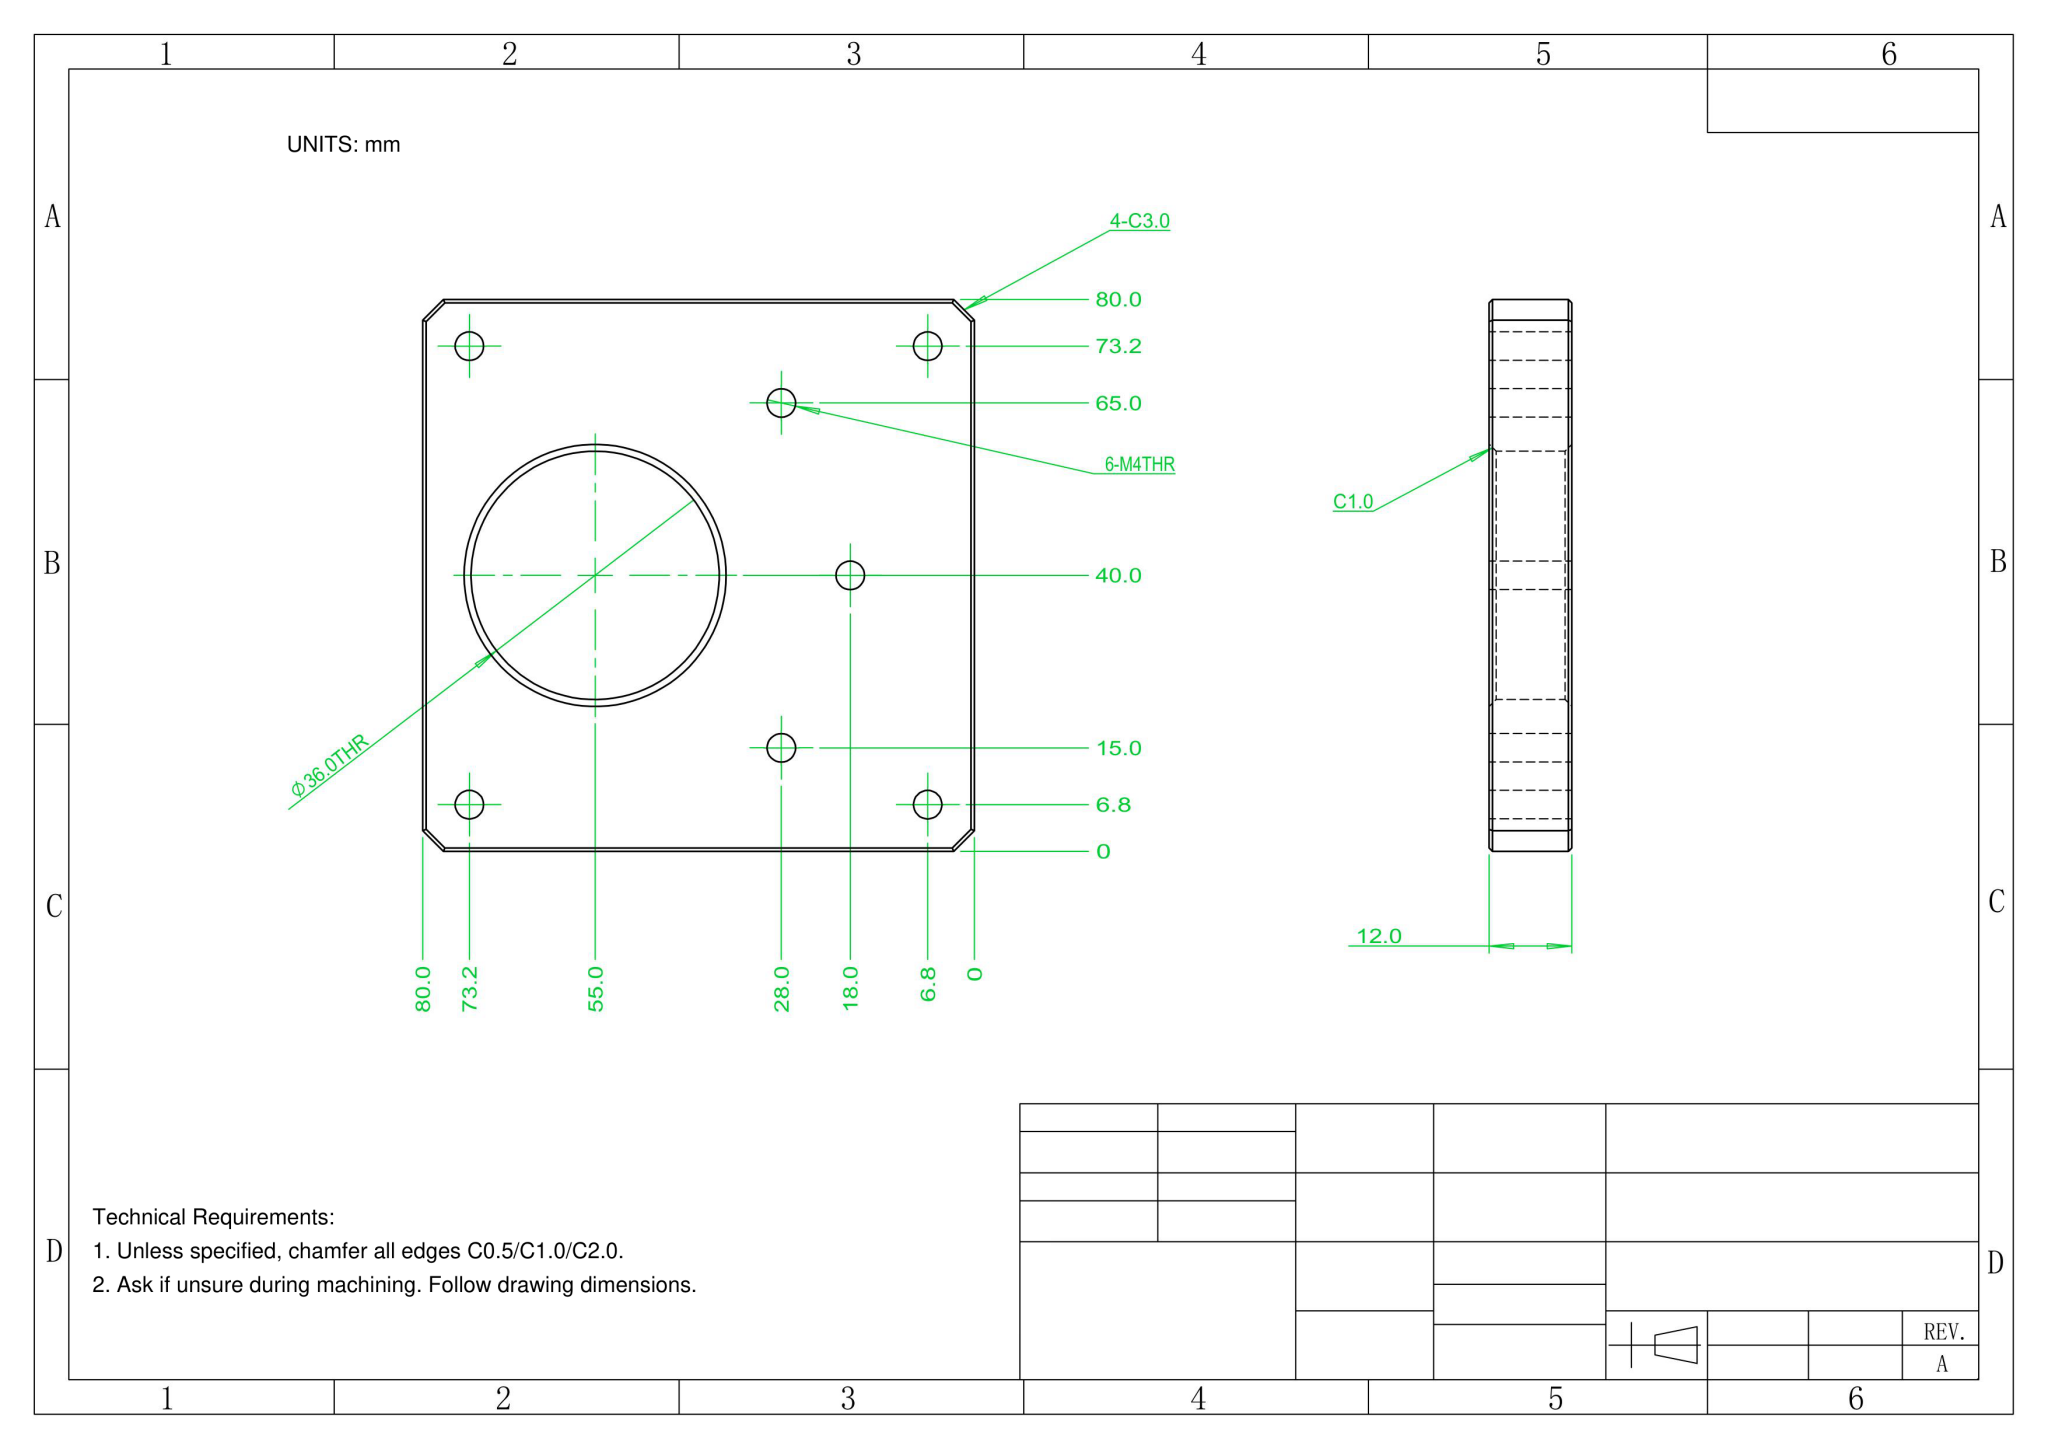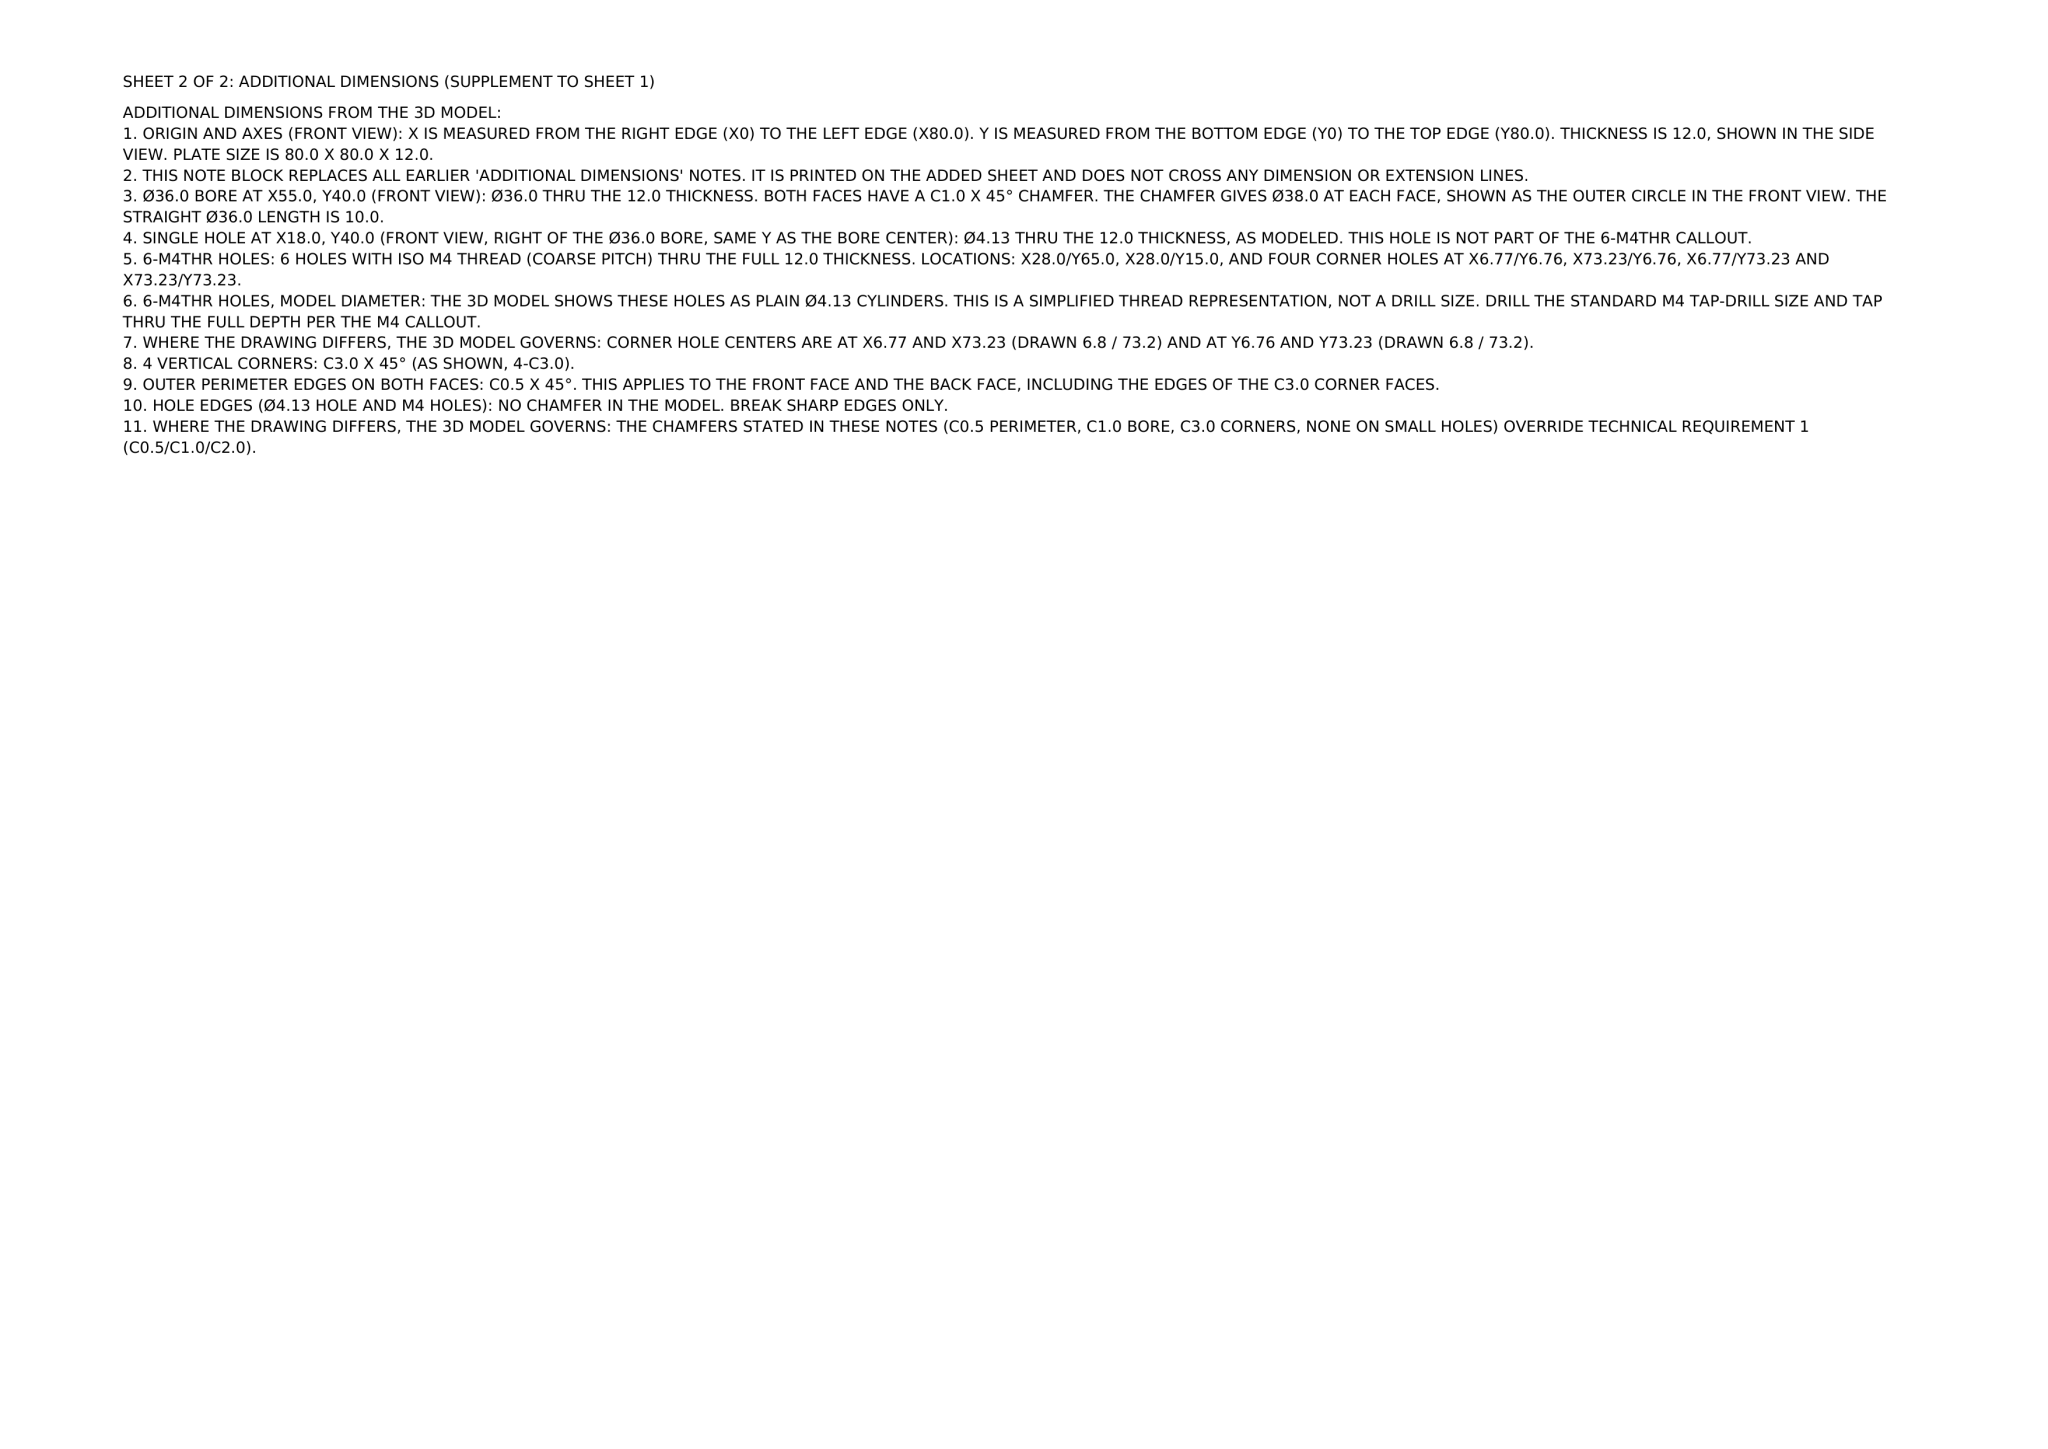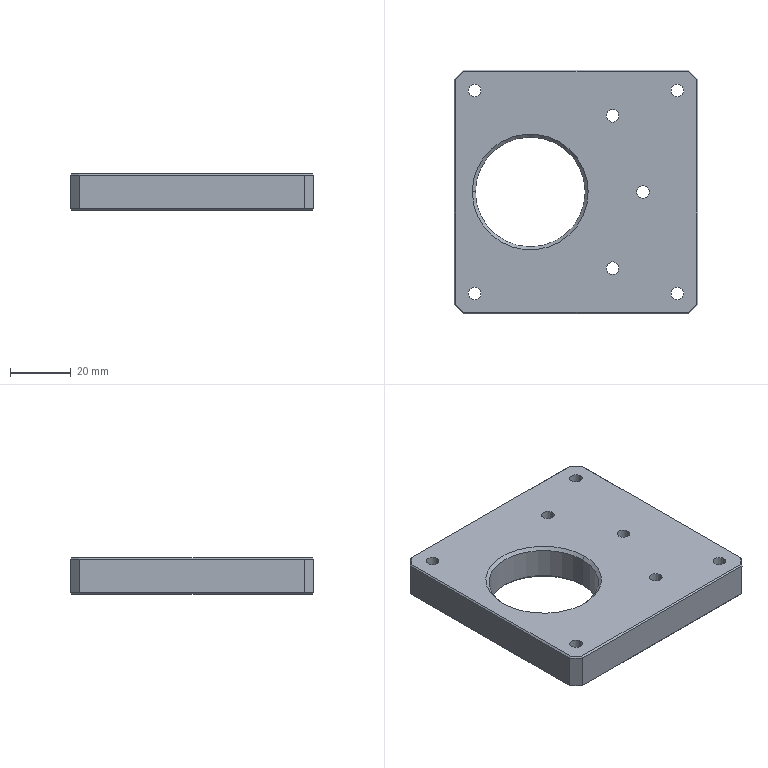Part | NX | mm | 1 solid | 46 faces | box 80 x 80 x 12 mm | volume 63049 mm3 | plane 26 | cylinder 16 | cone 4 | commonest cylinder face diameters 4.134 x14 36 x2